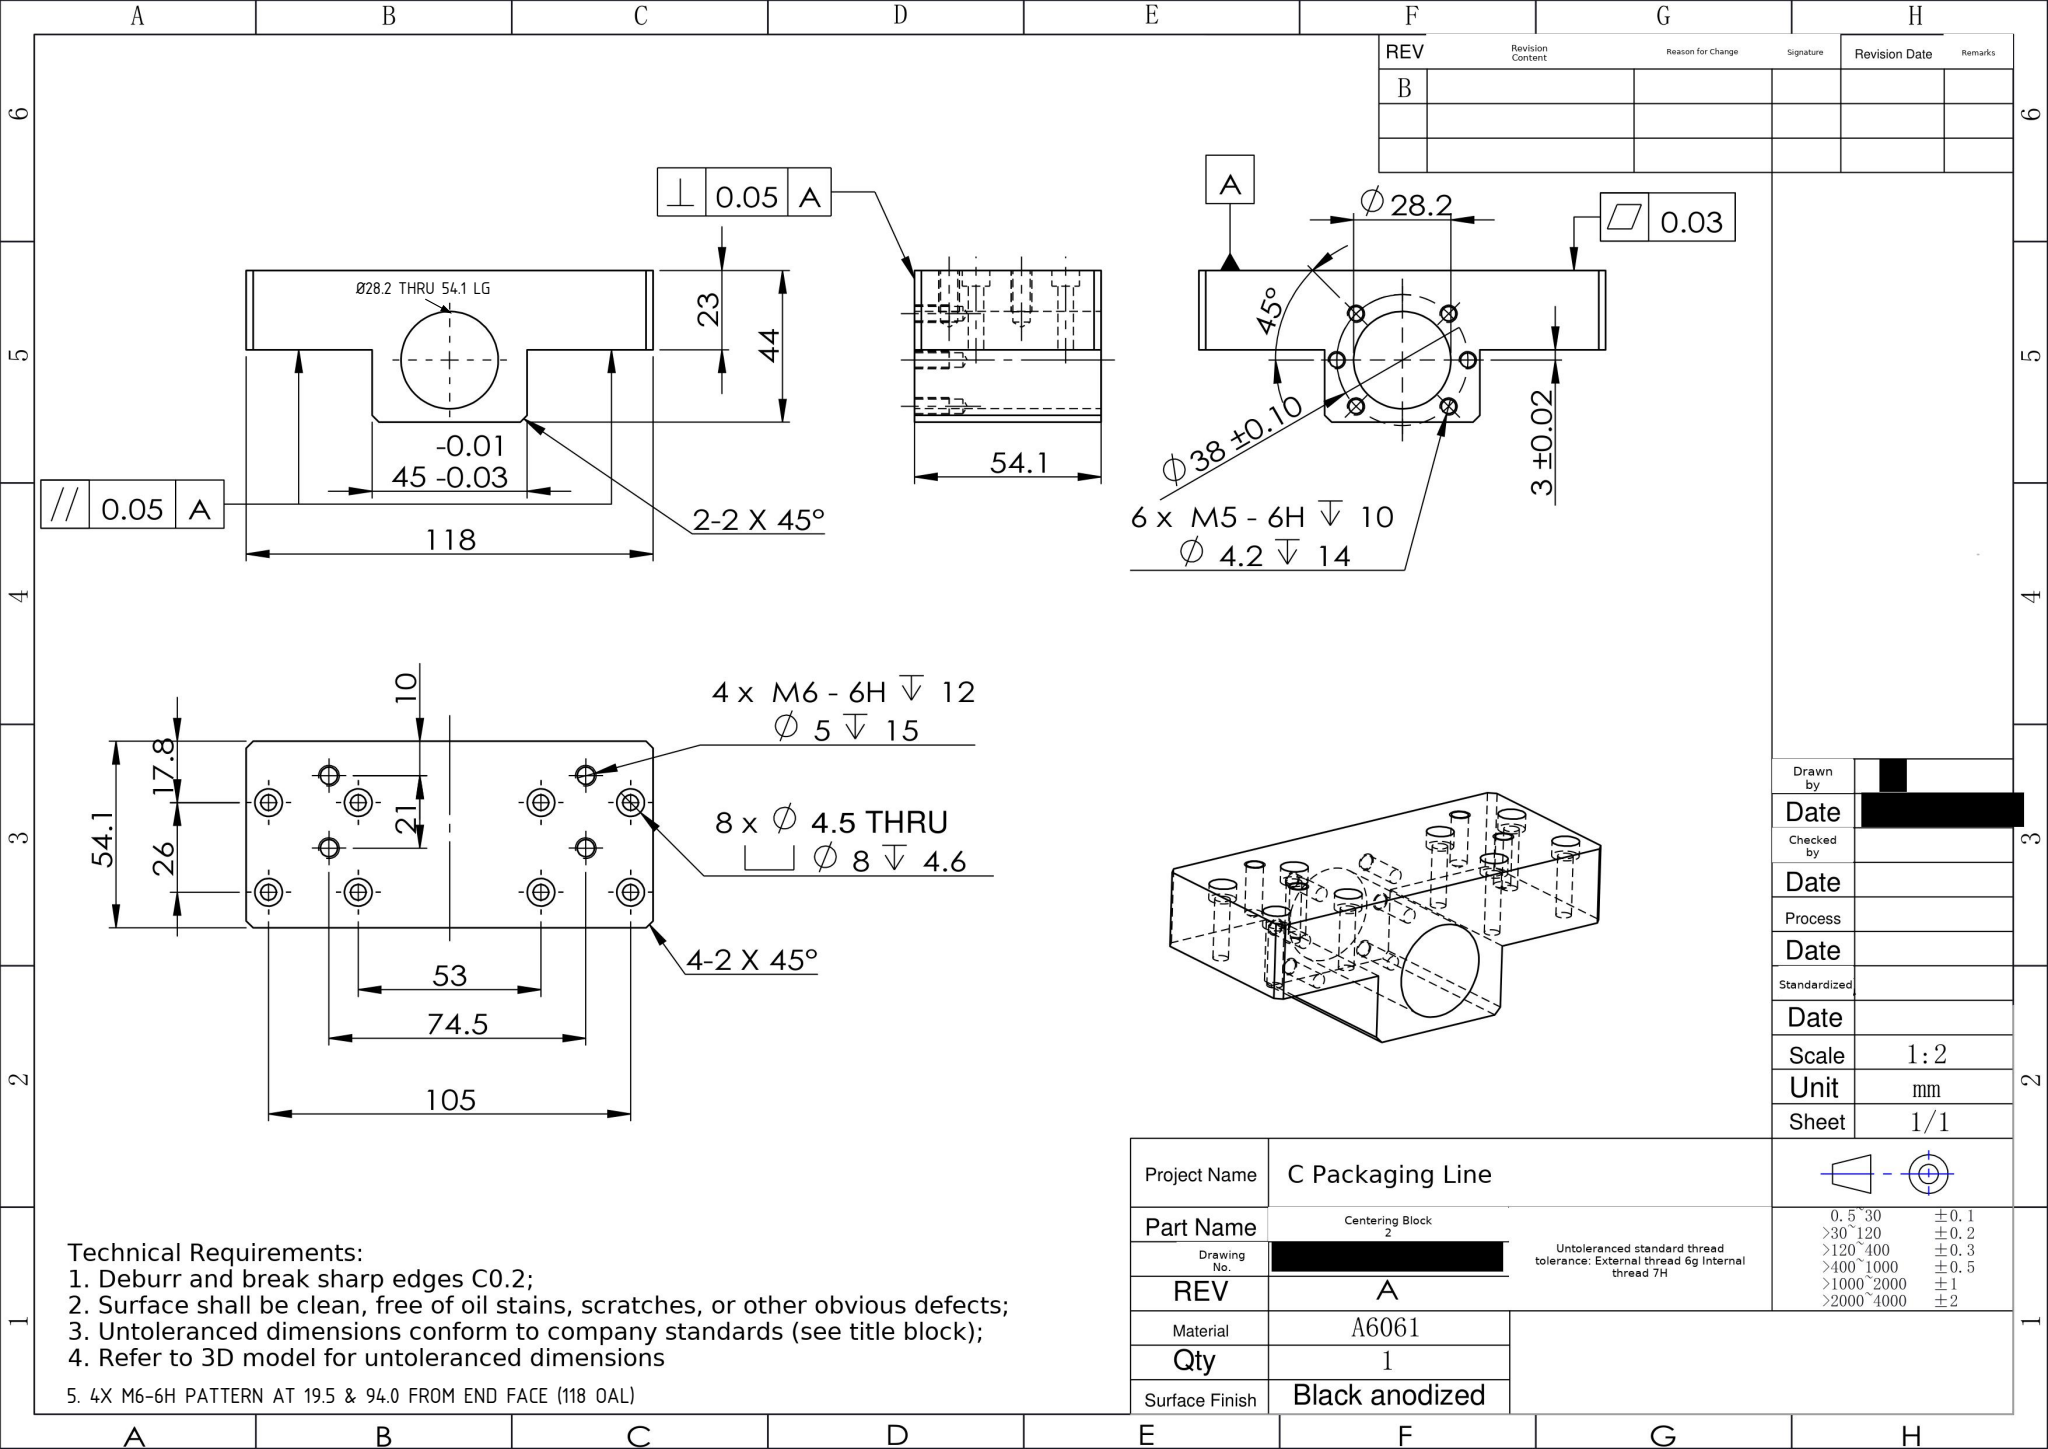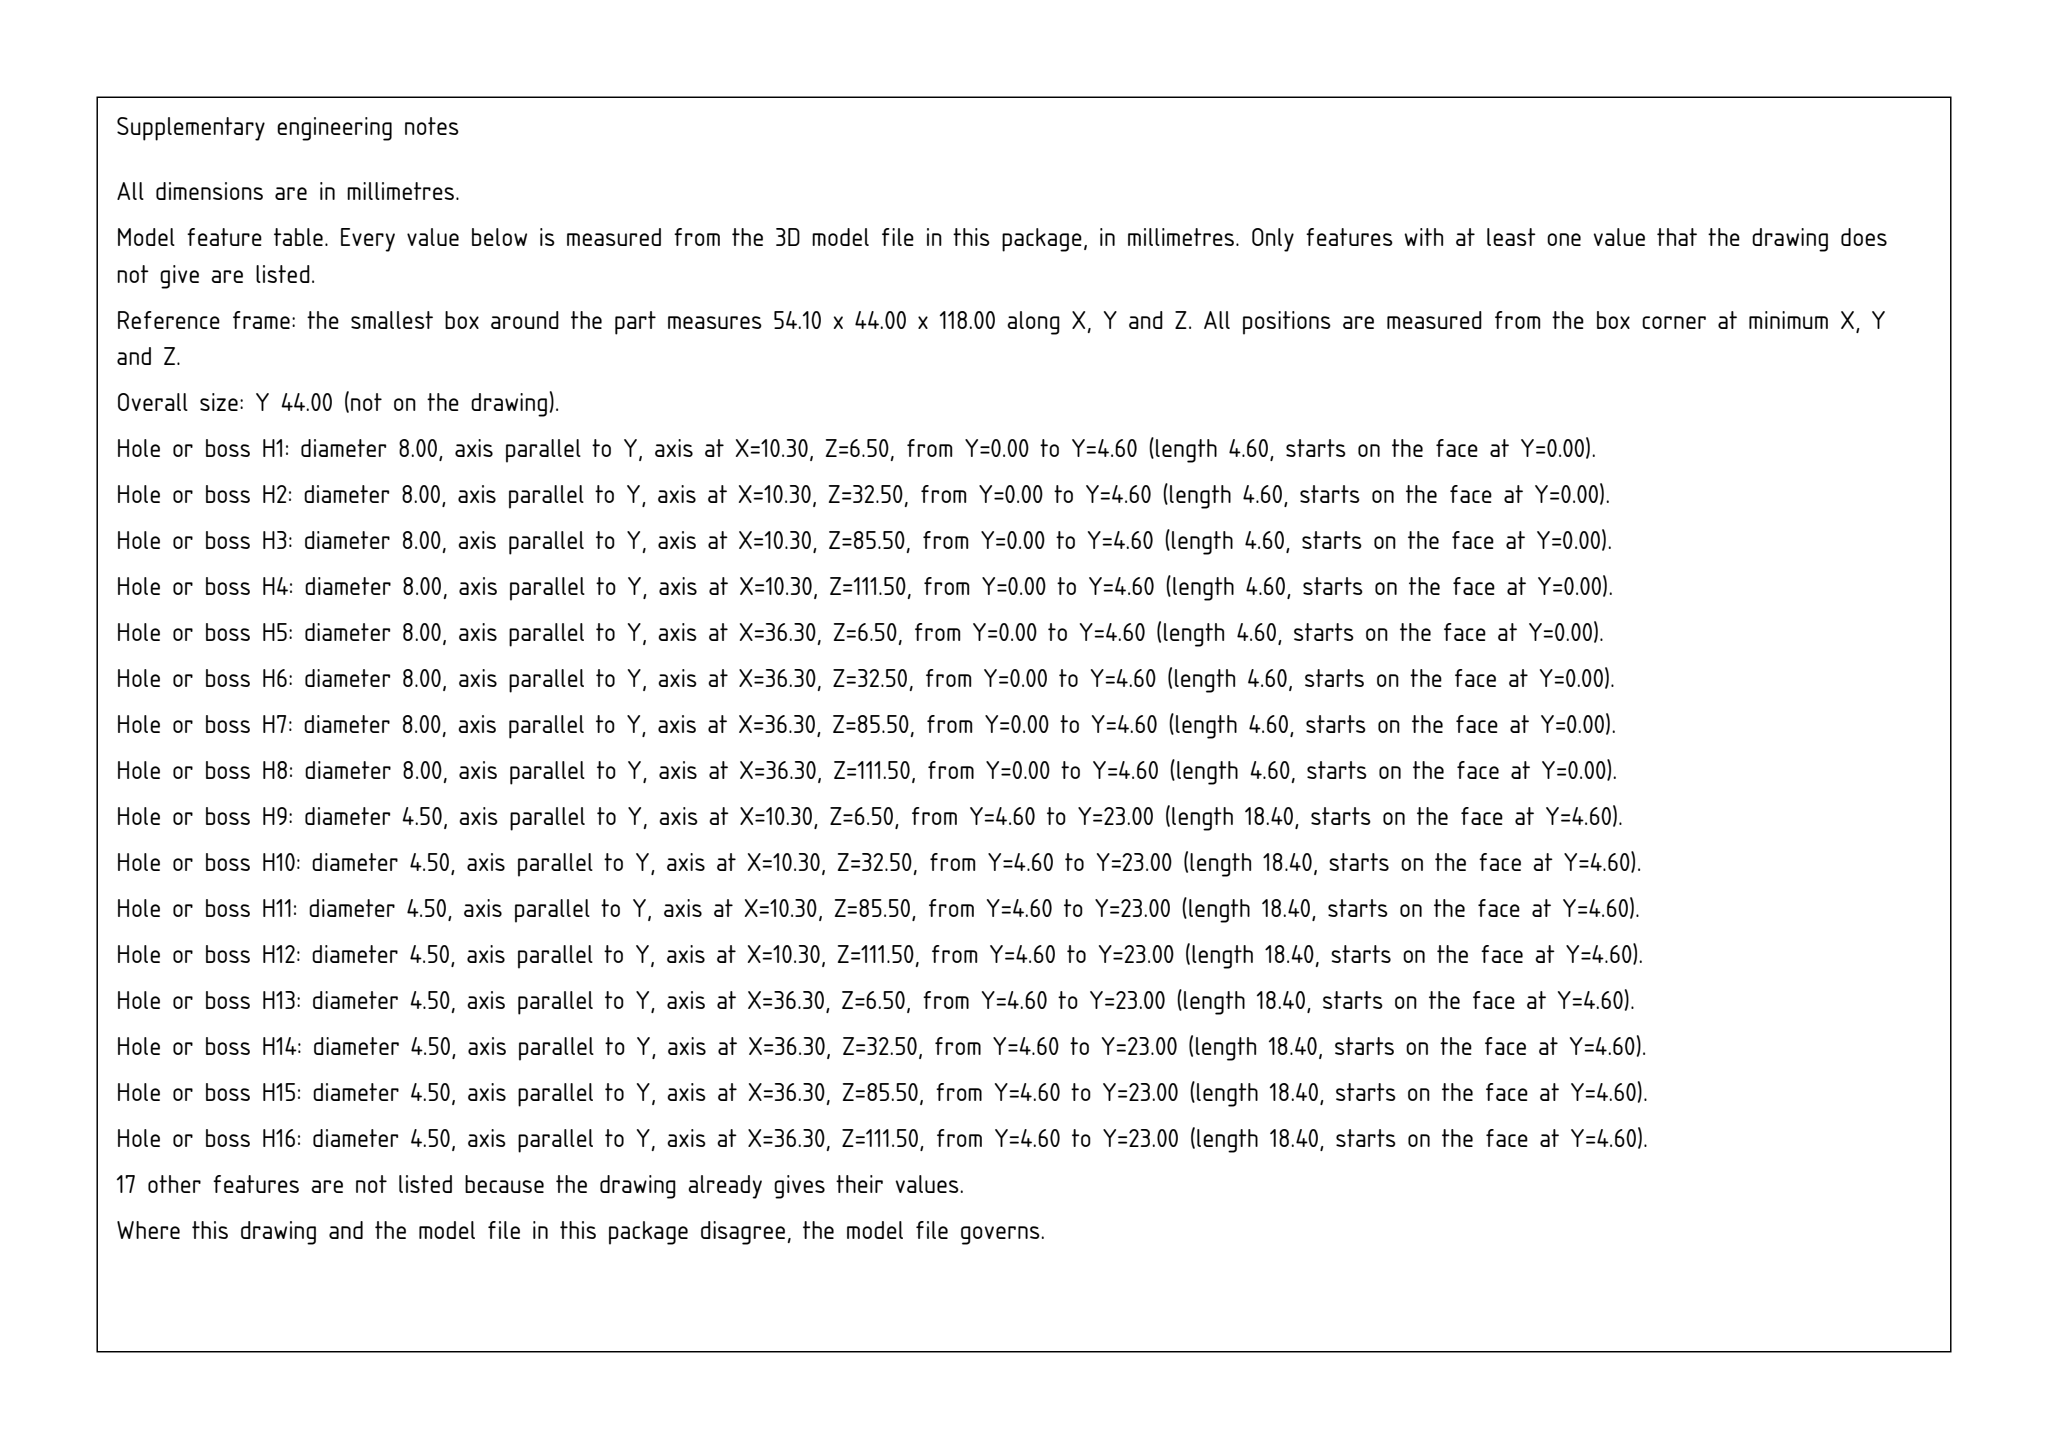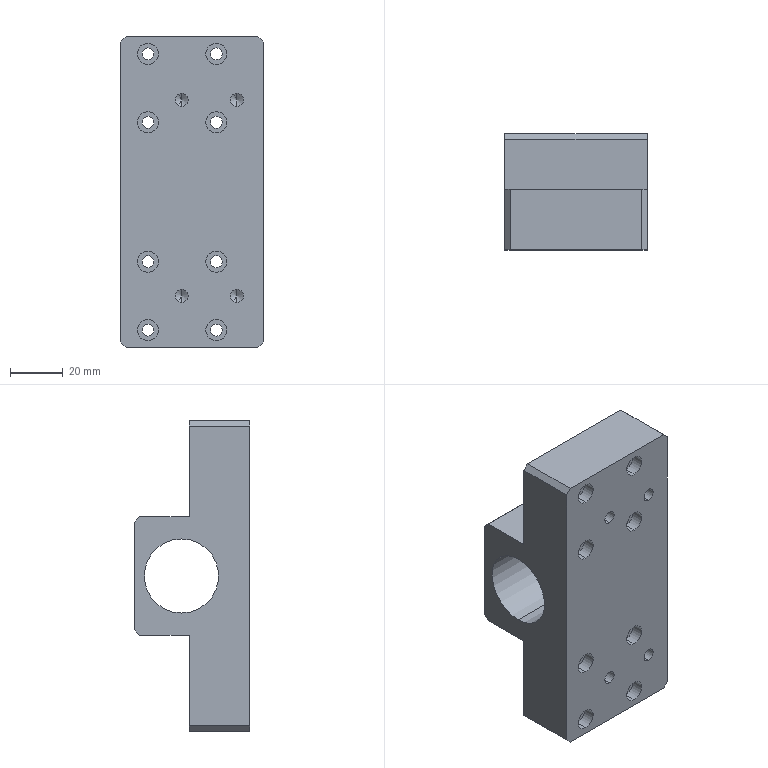Part | SolidWorks | mm | material A6061 | 1 solid | 98 faces | box 54.1 x 44 x 118 mm | volume 157155 mm3 | cylinder 54 | plane 24 | cone 20 | commonest cylinder face diameters 8 x16 4.5 x16 4.2 x12 5 x8 28.2 x2
Drawing notes:
Ø28.2 BORE THRU 54.1 LG, CL 26 ABOVE BOTTOM FACE (18 BELOW TOP FACE) | from the solid: cyl dia 28.2 axis x, length 54.1 = full bbox X, axis at y=26.0 of 44.0 bbox height
4X M6-6H PATTERN AT 19.5 & 94.0 FROM END FACE (118 OAL) | from the solid: Ø5.0 y-axis cyls at z=19.5 and z=94.0; bbox z=118.0
build123d program:
from build123d import *

# Parameters (mm, degrees)
SKETCH1_W                                       = 54.1
SKETCH1_H                                       = 118
BOSS_EXTRUDE1_DEPTH                             = 44
CUT_EXTRUDE2_DEPTH                              = 92.344
CUT_EXTRUDE2_DEPTH_BACK                         = 92.344
SKETCH3_R                                       = 14.1
SKETCH15_W                                      = 73
SKETCH15_H                                      = 42
CUT_EXTRUDE4_DEPTH                              = 92.344
M4_HEX_SOCKET_HEAD_CAP_SCREW_CBORE1_D           = 4.5
M4_HEX_SOCKET_HEAD_CAP_SCREW_CBORE1_CBORE_D     = 8
M4_HEX_SOCKET_HEAD_CAP_SCREW_CBORE1_CBORE_DEPTH = 4.6
CHAMFER1_SIZE                                   = 2
M6_TAPPED_HOLE3_D                               = 5
M6_TAPPED_HOLE3_DEPTH                           = 15
M6_TAPPED_HOLE3_TIP                             = 1.502
M5_TAPPED_HOLE1_AT_2_COUNT                      = 2
M5_TAPPED_HOLE1_AT_2_PITCH                      = 38
CIRPATTERN1_COUNT                               = 2
CIRPATTERN1_ANGLE                               = 45
CIRPATTERN1_THE_OTHER_WAY_COUNT                 = 2
CIRPATTERN1_THE_OTHER_WAY_ANGLE                 = 45


with BuildPart() as part:
    # Sketch1 → Boss-Extrude1 (new body)
    with BuildSketch(Plane(origin=(0, 0, 0), x_dir=(1, 0, 0), z_dir=(0, 1, 0))):
        Rectangle(SKETCH1_W, SKETCH1_H)
    extrude(amount=BOSS_EXTRUDE1_DEPTH)

    # Sketch3 → Cut-Extrude2 (cut, two sides: drawn at the far end of the back side and taken through both)
    with BuildSketch(Plane(origin=(27.05, 0, 0), x_dir=(0, 0, -1), z_dir=(1, 0, 0)).offset(-CUT_EXTRUDE2_DEPTH_BACK)):
        with Locations((0, 26)):
            Circle(SKETCH3_R)
    extrude(amount=CUT_EXTRUDE2_DEPTH + CUT_EXTRUDE2_DEPTH_BACK, mode=Mode.SUBTRACT)

    # Sketch15 → Cut-Extrude4 (cut, through all)
    with BuildSketch(Plane(origin=(27.05, 0, 0), x_dir=(0, 0, -1), z_dir=(1, 0, 0))):
        with Locations((-59, 44)):
            Rectangle(SKETCH15_W, SKETCH15_H)
        with Locations((59, 44)):
            Rectangle(SKETCH15_W, SKETCH15_H)
    extrude(amount=-CUT_EXTRUDE4_DEPTH, mode=Mode.SUBTRACT)

    # M4 Hex Socket Head Cap Screw CBORE1 (through all)
    with Locations(Plane(origin=(0, 0, 0), x_dir=(-1, 0, 0), z_dir=(0, -1, 0))):
        with Locations((16.75, 26.5), (-9.25, 26.5), (16.75, 52.5), (-9.25, 52.5), (16.75, -26.5), (-9.25, -26.5), (-9.25, -52.5), (16.75, -52.5)):
            CounterBoreHole(M4_HEX_SOCKET_HEAD_CAP_SCREW_CBORE1_D / 2, M4_HEX_SOCKET_HEAD_CAP_SCREW_CBORE1_CBORE_D / 2, M4_HEX_SOCKET_HEAD_CAP_SCREW_CBORE1_CBORE_DEPTH)

    # Chamfer1
    chamfer1_edges = [part.edges().sort_by_distance(p)[0] for p in [
        (0, 44, -22.5),
        (0, 44, 22.5),
        (-27.05, 11.5, -59),
        (27.05, 11.5, -59),
        (27.05, 11.5, 59),
        (-27.05, 11.5, 59),
    ]]
    chamfer(chamfer1_edges, length=CHAMFER1_SIZE)

    # M6 Tapped Hole3
    with Locations(Plane(origin=(0, 0, 0), x_dir=(-1, 0, 0), z_dir=(0, -1, 0))):
        with Locations((-17.05, -35), (-17.05, 39.5), (3.95, 39.5), (3.95, -35)):
            Hole(M6_TAPPED_HOLE3_D / 2, depth=M6_TAPPED_HOLE3_DEPTH)
            with Locations((0, 0, -(M6_TAPPED_HOLE3_DEPTH + M6_TAPPED_HOLE3_TIP / 2))):  # 118° drill point
                Cone(0, M6_TAPPED_HOLE3_D / 2, M6_TAPPED_HOLE3_TIP, mode=Mode.SUBTRACT)

    # Sketch29 → M5 Tapped Hole1 (revolve, cut)
    with BuildSketch(Plane(origin=(27.05, 26, 19), x_dir=(0, 0, -1), z_dir=(0, 1, 0))):
        Polygon((0, 0), (0, 15.262), (2.1, 14), (2.1, 0), align=None)
    m5_tapped_hole1 = revolve(axis=Axis((33.4, 26, 19), (-1, 0, 0)), mode=Mode.SUBTRACT)

    # M5 Tapped Hole1 at 2: M5 Tapped Hole1 ×2
    with Locations(*[(0, 0, -i * M5_TAPPED_HOLE1_AT_2_PITCH) for i in range(1, M5_TAPPED_HOLE1_AT_2_COUNT)]):
        add(m5_tapped_hole1, mode=Mode.SUBTRACT)

    # CirPattern1: M5 Tapped Hole1 ×2 about axis
    cirpattern1_axis = Axis((0, 26, 0), (-1, 0, 0))
    for i in range(1, CIRPATTERN1_COUNT):
        add(m5_tapped_hole1.rotate(cirpattern1_axis, i * CIRPATTERN1_ANGLE / (CIRPATTERN1_COUNT - 1)), mode=Mode.SUBTRACT)

    # CirPattern1 copy 1 sketch → CirPattern1 copy 1 (revolve, cut)
    with BuildSketch(Plane(origin=(27.05, 12.565, -13.435), x_dir=(0, -0.7071, -0.7071), z_dir=(0, 0.7071, -0.7071))):
        Polygon((0, 0), (0, 15.262), (2.1, 14), (2.1, 0), align=None)
    revolve(axis=Axis((33.4, 12.565, -13.435), (-1, 0, 0)), mode=Mode.SUBTRACT)

    # CirPattern1 the other way: M5 Tapped Hole1 ×2 about axis
    cirpattern1_the_other_way_axis = Axis((0, 26, 0), (1, 0, 0))
    for i in range(1, CIRPATTERN1_THE_OTHER_WAY_COUNT):
        add(m5_tapped_hole1.rotate(cirpattern1_the_other_way_axis, i * CIRPATTERN1_THE_OTHER_WAY_ANGLE / (CIRPATTERN1_THE_OTHER_WAY_COUNT - 1)), mode=Mode.SUBTRACT)

    # CirPattern1 the other way copy 1 sketch → CirPattern1 the other way copy 1 (revolve, cut)
    with BuildSketch(Plane(origin=(27.05, 39.435, -13.435), x_dir=(0, 0.7071, -0.7071), z_dir=(0, 0.7071, 0.7071))):
        Polygon((0, 0), (0, 15.262), (2.1, 14), (2.1, 0), align=None)
    revolve(axis=Axis((33.4, 39.435, -13.435), (-1, 0, 0)), mode=Mode.SUBTRACT)


solid = part.part